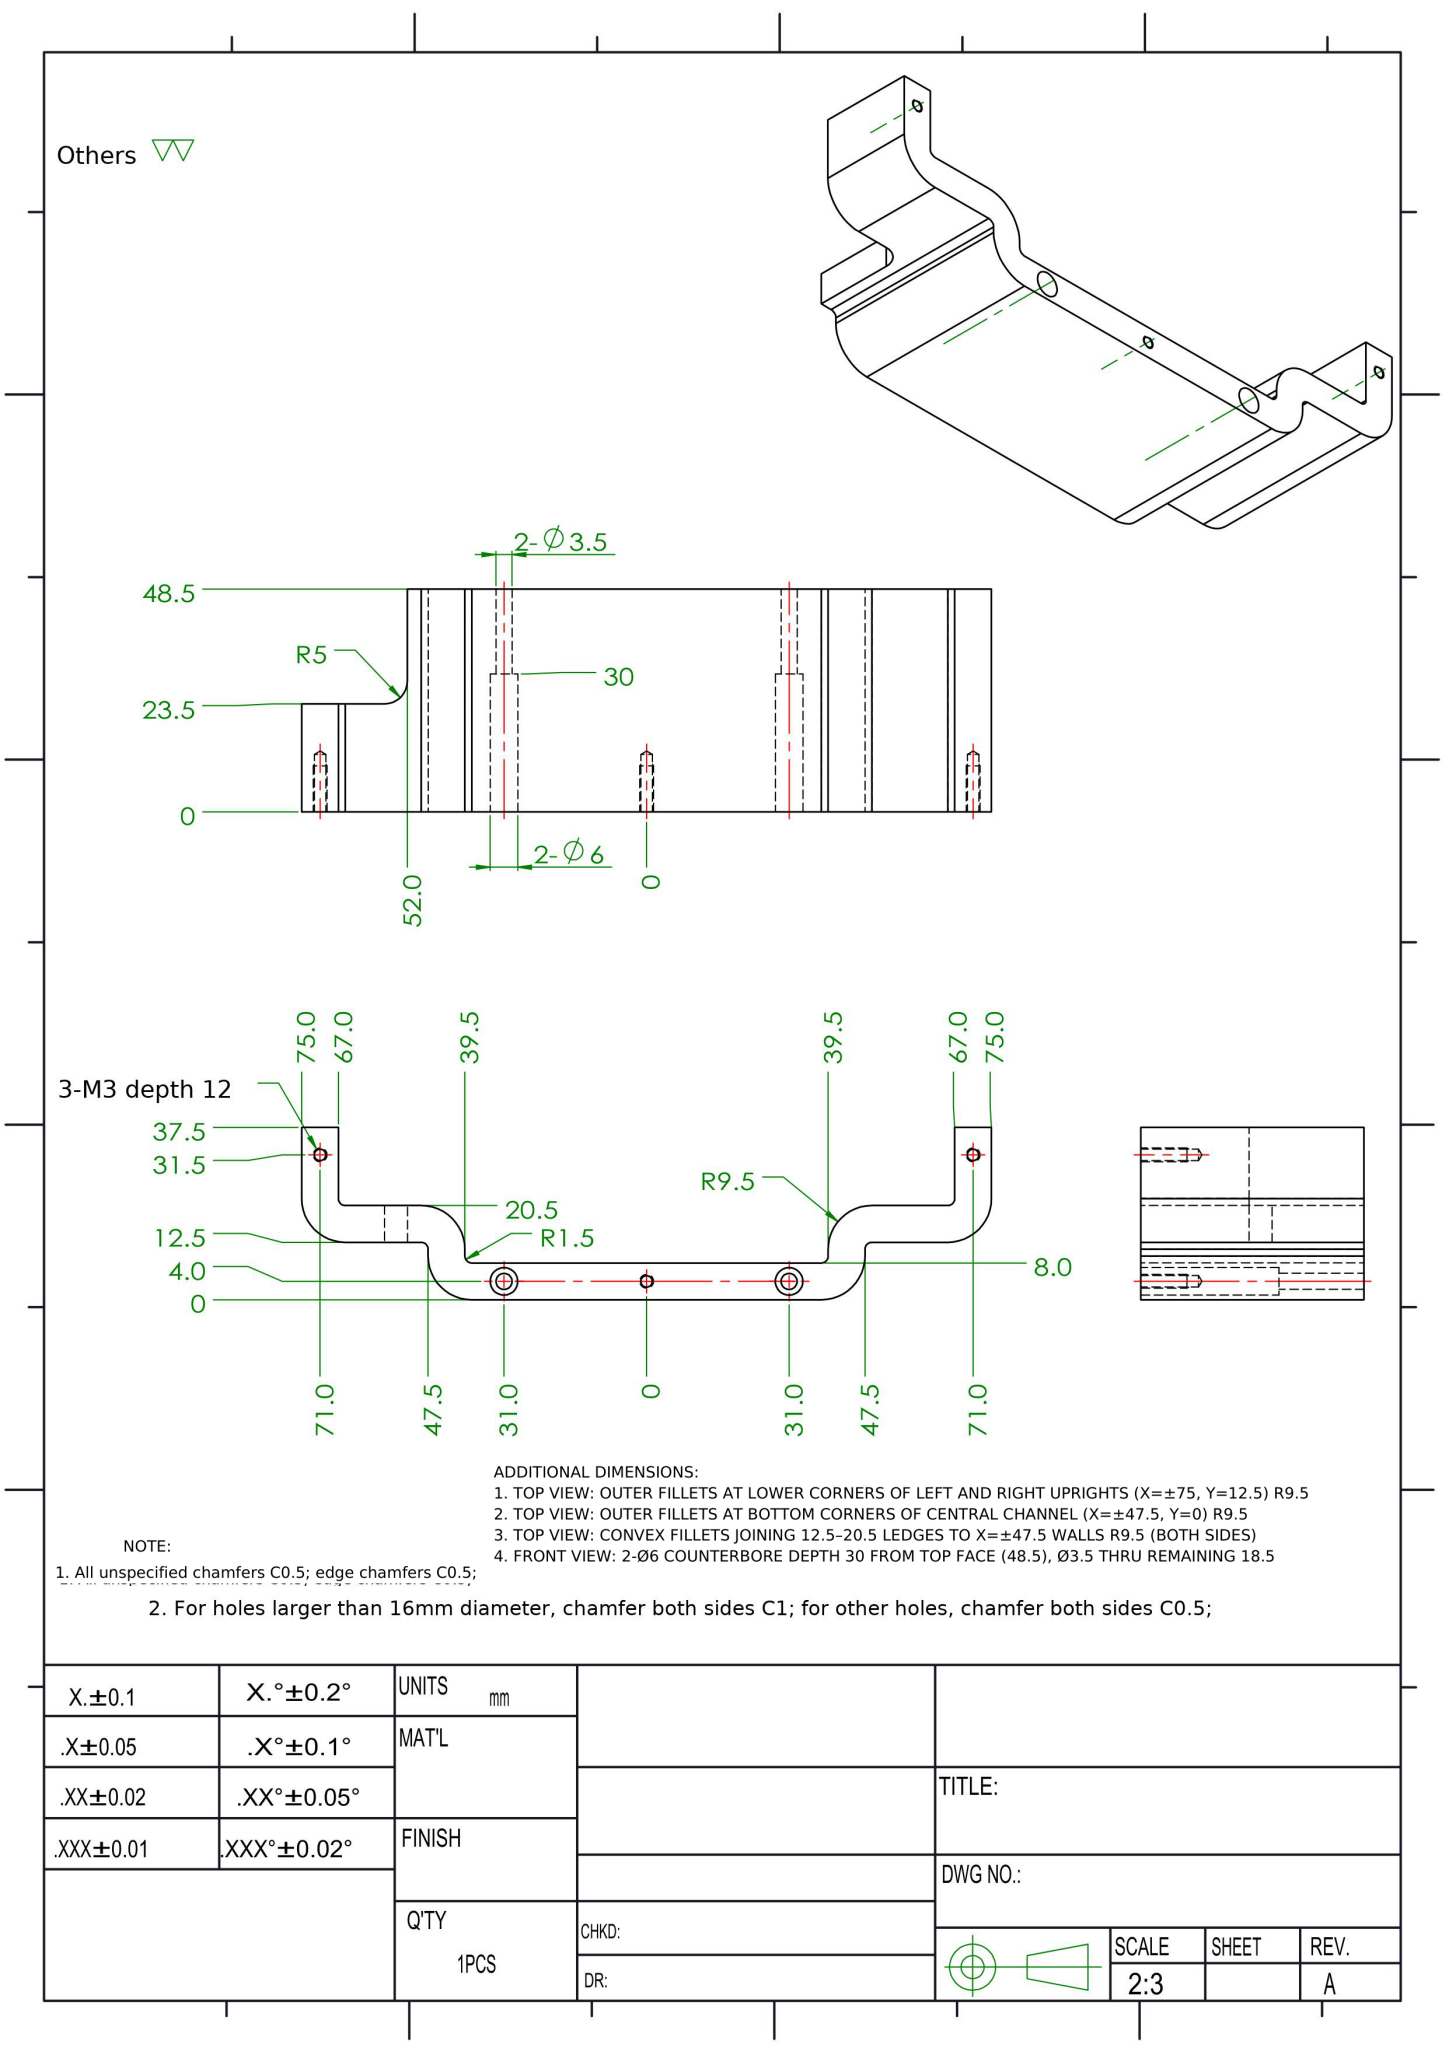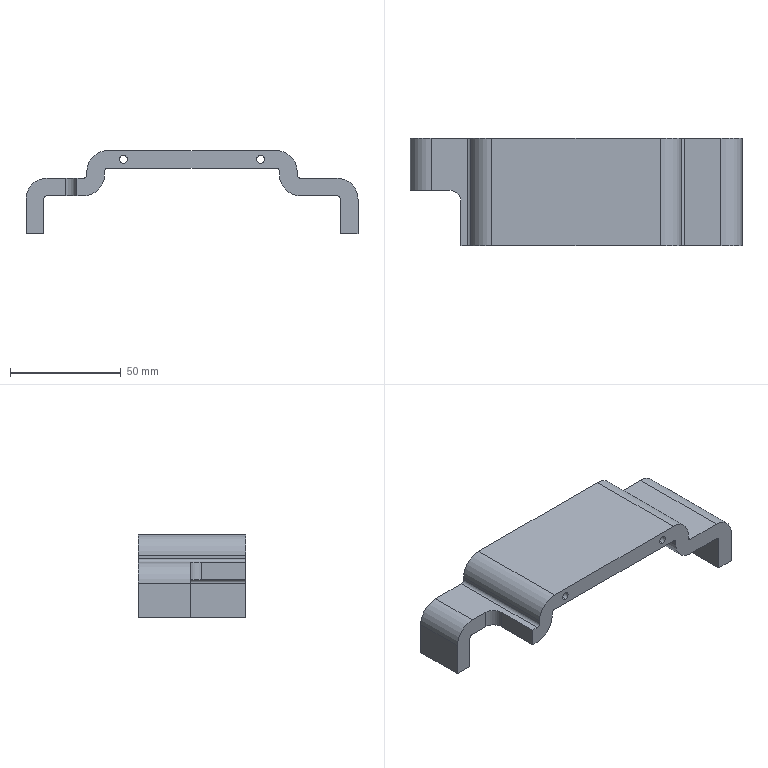Part | NX | mm | 1 solid | 55 faces | box 150 x 48.5 x 37.5 mm | volume 65871 mm3 | cylinder 27 | plane 22 | cone 6 | commonest cylinder face diameters 2.5 x6 3 x6 19 x6 6 x4 3.5 x4 10 x1